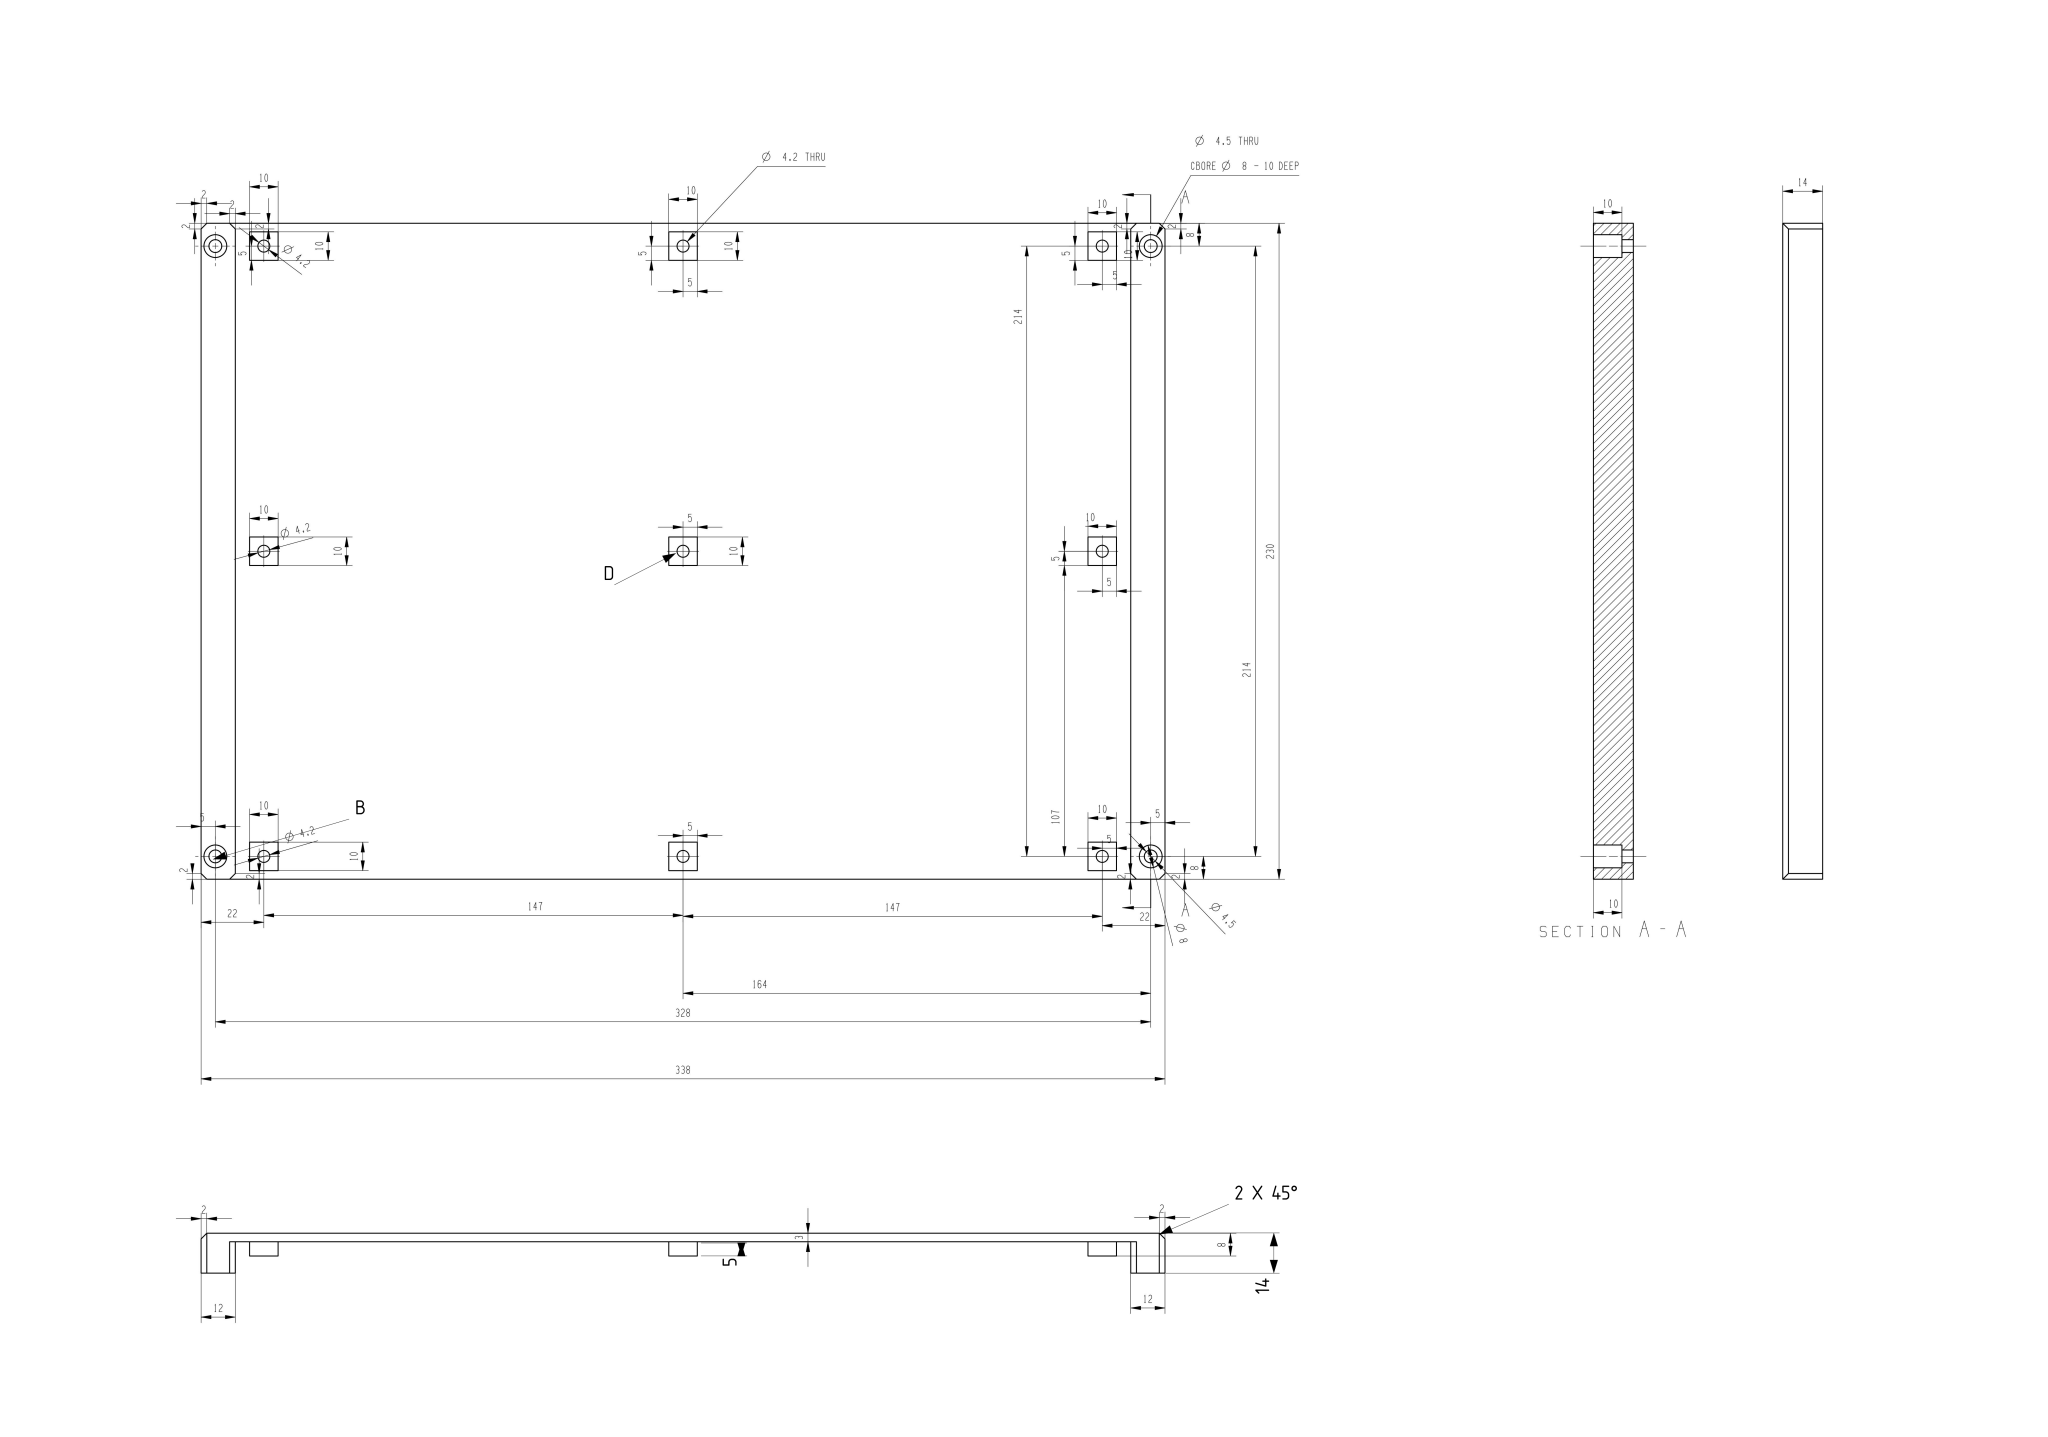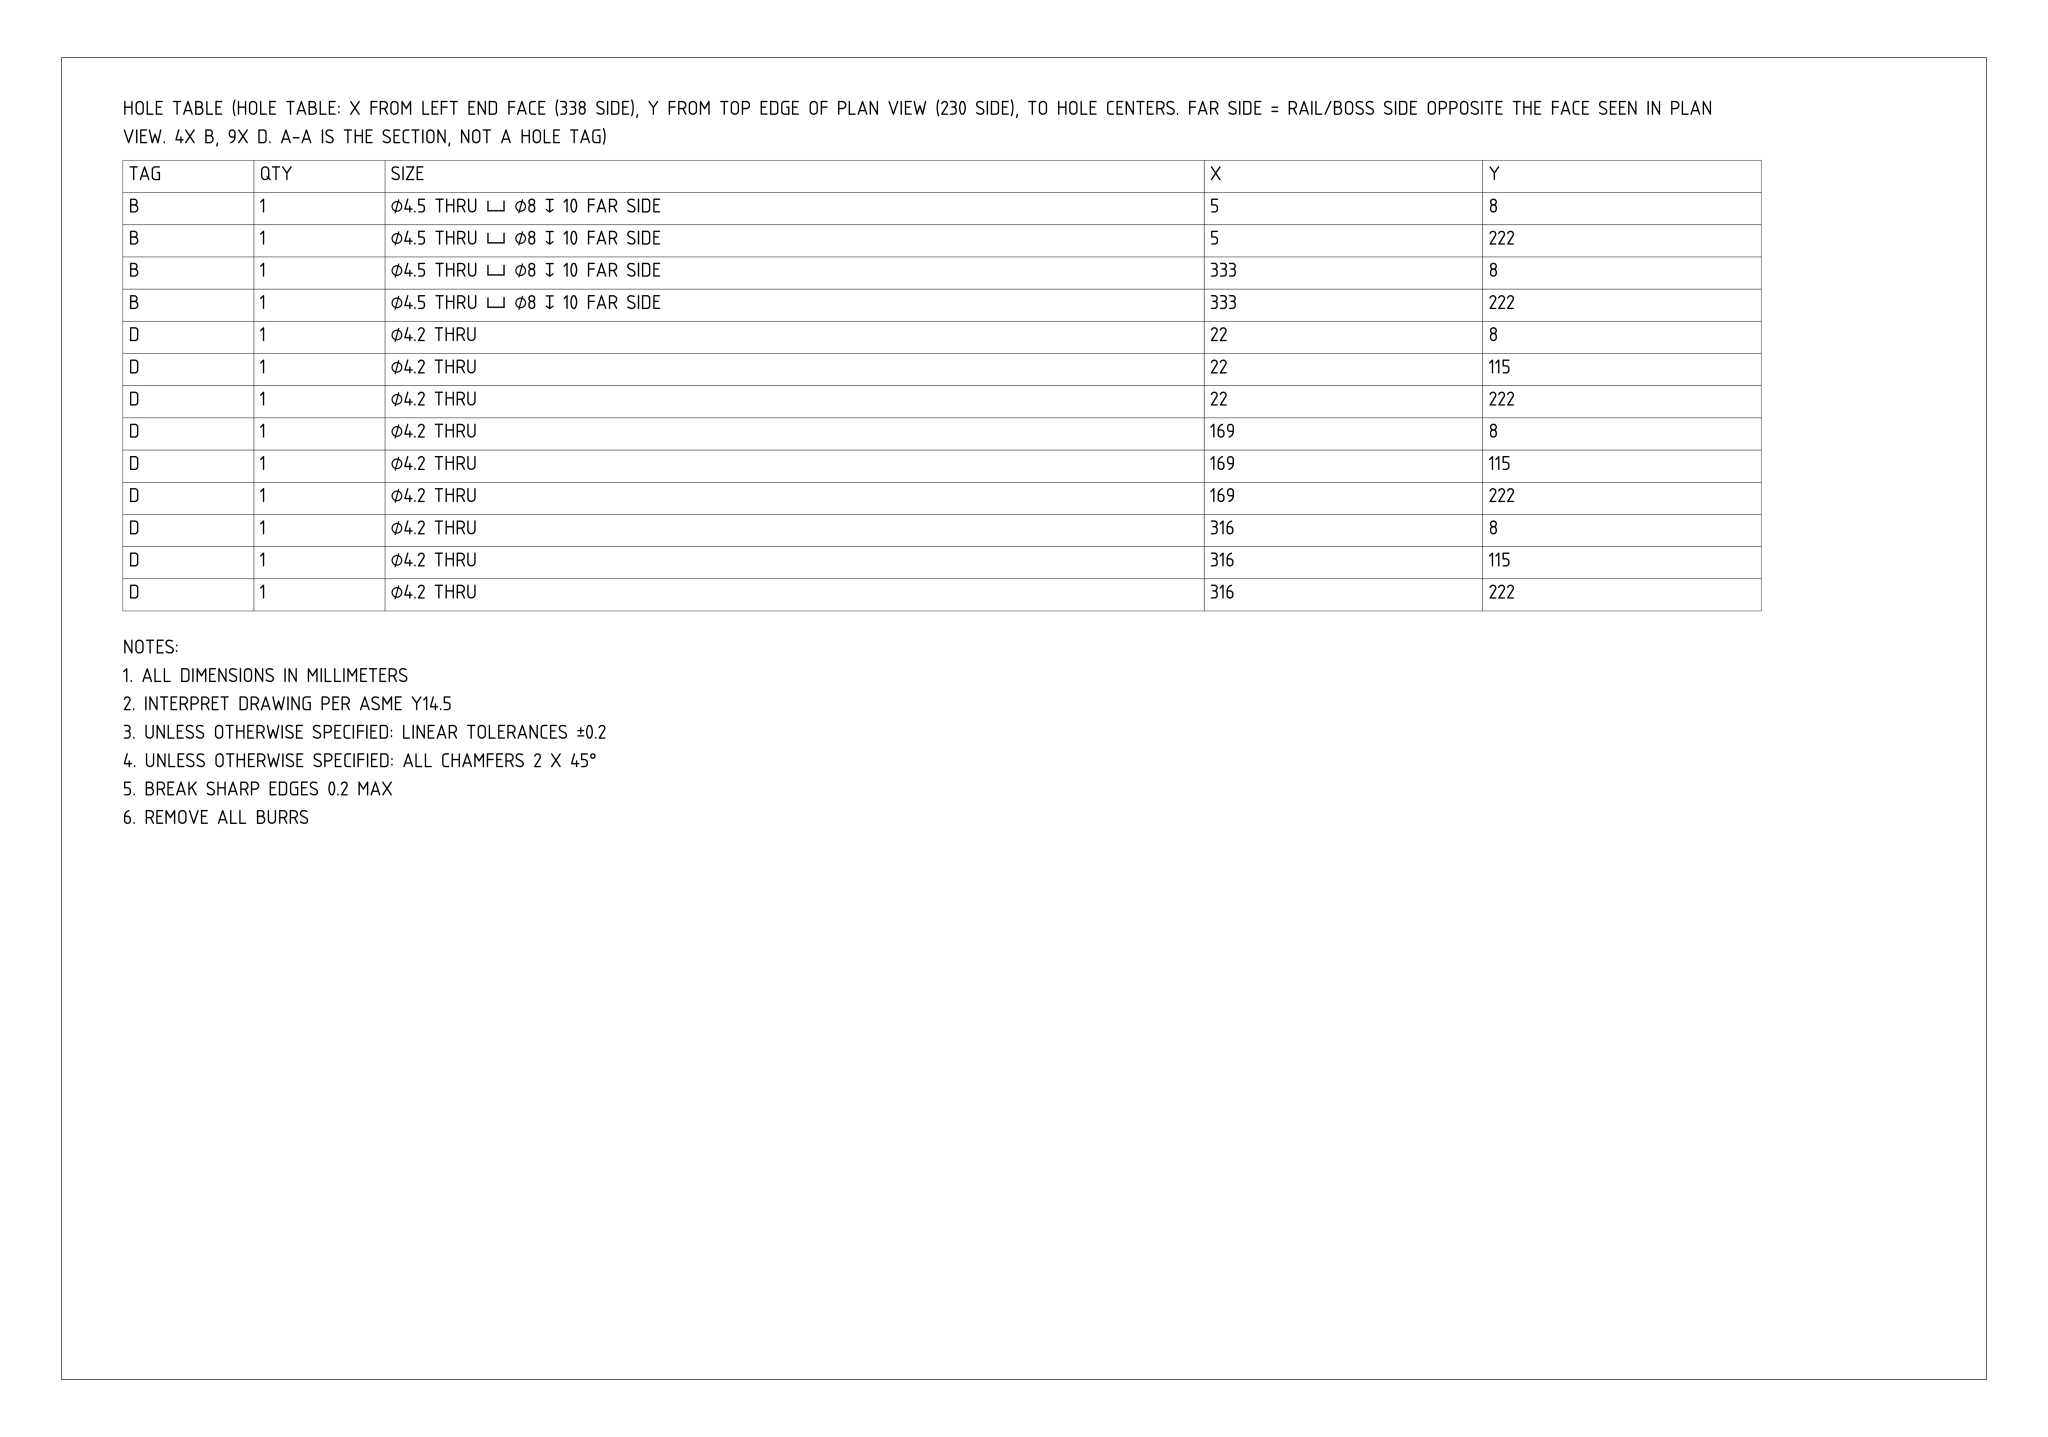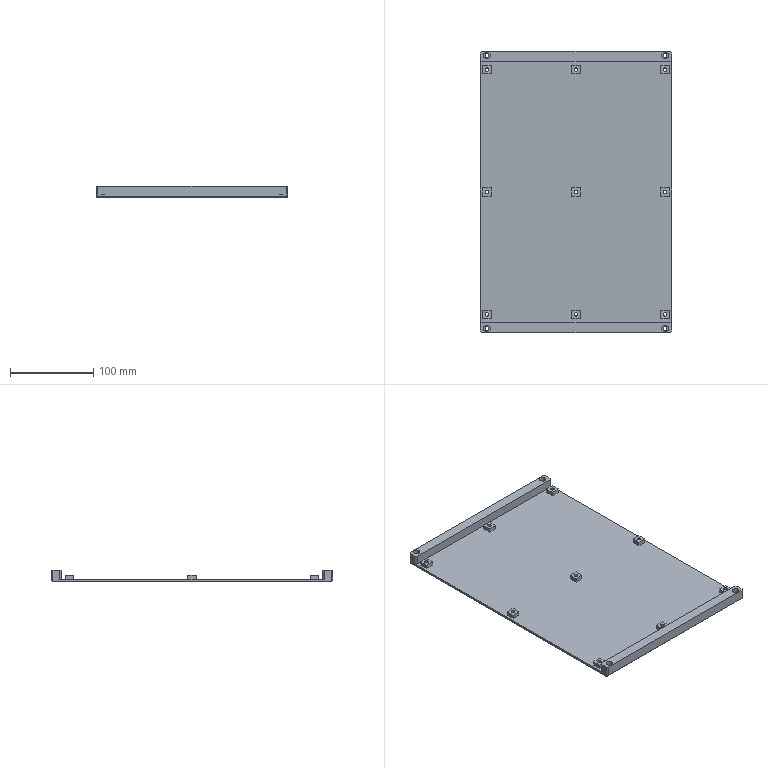Part | NX | mm | 1 solid | 86 faces | box 230 x 338 x 14 mm | volume 294068 mm3 | plane 69 | cylinder 17 | commonest cylinder face diameters 4.2 x9 4.5 x4 8 x4